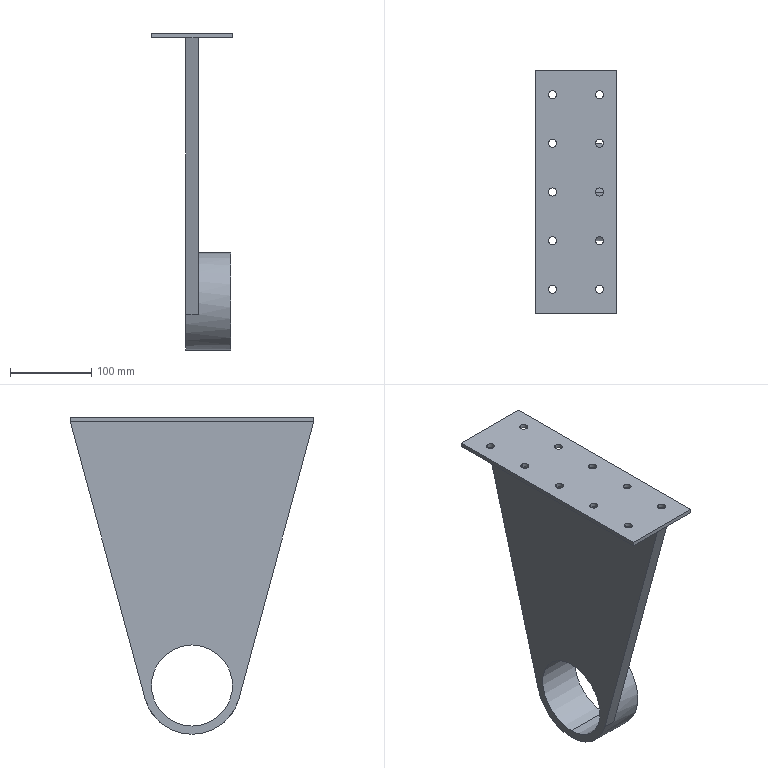Component | SolidWorks | BrushRollerHolder-1 | 1 solid | 36 faces | box 100 x 300 x 390 mm | volume 1352677 mm3 | cylinder 24 | plane 12 | commonest cylinder face diameters 10 x20 100 x2 120 x2
build123d program:
from build123d import *

# Parameters (mm, degrees)
SKETCH1_W                = 300
SKETCH1_H                = 100
BOSS_EXTRUDE1_DEPTH      = 5
BOSS_EXTRUDE2_DEPTH      = 8
BOSS_EXTRUDE2_DEPTH_BACK = 8
SKETCH4_R                = 50
BOSS_EXTRUDE3_START      = 40
SKETCH5_R                = 60
SKETCH5_R_2              = 50
BOSS_EXTRUDE3_DEPTH      = 40
SKETCH6_R                = 5
CUT_EXTRUDE2_DEPTH       = 40
LPATTERN1_COUNT          = 5
LPATTERN1_PITCH          = 60
MIRROR1_COPY_1_SKETCH_R  = 5
MIRROR1_COPY_1_DEPTH     = 40
MIRROR1_COPY_2_SKETCH_R  = 5
MIRROR1_COPY_2_DEPTH     = 40
MIRROR1_COPY_3_SKETCH_R  = 5
MIRROR1_COPY_3_DEPTH     = 40
MIRROR1_COPY_4_SKETCH_R  = 5
MIRROR1_COPY_4_DEPTH     = 40


with BuildPart() as part:
    # Sketch1 → Boss-Extrude1 (new body)
    with BuildSketch(Plane.XY):
        Rectangle(SKETCH1_W, SKETCH1_H)
    extrude(amount=BOSS_EXTRUDE1_DEPTH)

    # Sketch4 → Boss-Extrude2 (add, two sides: drawn at the far end of the back side and taken through both)
    with BuildSketch(Plane(origin=(0, 0, 0), x_dir=(1, 0, 0), z_dir=(0, 1, 0)).offset(-BOSS_EXTRUDE2_DEPTH_BACK)):
        with BuildLine():
            Line((-57.921, 340.656), (-150, 0))
            Line((-150, 0), (150, 0))
            Line((150, 0), (57.921, 340.656))
            ThreePointArc((57.921, 340.656), (0, 385), (-57.921, 340.656))
        make_face()
        with Locations(Location((0, 325, 0), (0, 0, 270))):
            Circle(SKETCH4_R, mode=Mode.SUBTRACT)
    extrude(amount=BOSS_EXTRUDE2_DEPTH + BOSS_EXTRUDE2_DEPTH_BACK)

    # Sketch5 → Boss-Extrude3 (add)
    with BuildSketch(Plane(origin=(0, -8, 0), x_dir=(-1, 0, 0), z_dir=(0, -1, 0)).offset(BOSS_EXTRUDE3_START)):
        with Locations(Location((0, 325, 0), (0, 0, 15.125))):
            Circle(SKETCH5_R)
        with Locations(Location((0, 325, 0), (0, 0, 270))):
            Circle(SKETCH5_R_2, mode=Mode.SUBTRACT)
    extrude(amount=-BOSS_EXTRUDE3_DEPTH)

    # Sketch6 → Cut-Extrude2 (cut)
    with BuildSketch(Plane(origin=(0, 0, 0), x_dir=(-1, 0, 0), z_dir=(0, 0, -1))):
        with Locations((-120, 29)):
            Circle(SKETCH6_R)
    cut_extrude2 = extrude(amount=-CUT_EXTRUDE2_DEPTH, mode=Mode.SUBTRACT)

    # LPattern1: Cut-Extrude2 ×5
    with Locations(*[(-i * LPATTERN1_PITCH, 0, 0) for i in range(1, LPATTERN1_COUNT)]):
        add(cut_extrude2, mode=Mode.SUBTRACT)

    # Mirror1: Cut-Extrude2 across plane
    add(cut_extrude2.mirror(Plane.ZX), mode=Mode.SUBTRACT)

    # Mirror1 copy 1 sketch → Mirror1 copy 1 (cut)
    with BuildSketch(Plane(origin=(-60, 0, 0), x_dir=(-1, 0, 0), z_dir=(0, 0, -1))):
        with Locations((-120, -29)):
            Circle(MIRROR1_COPY_1_SKETCH_R)
    extrude(amount=-MIRROR1_COPY_1_DEPTH, mode=Mode.SUBTRACT)

    # Mirror1 copy 2 sketch → Mirror1 copy 2 (cut)
    with BuildSketch(Plane(origin=(-120, 0, 0), x_dir=(-1, 0, 0), z_dir=(0, 0, -1))):
        with Locations((-120, -29)):
            Circle(MIRROR1_COPY_2_SKETCH_R)
    extrude(amount=-MIRROR1_COPY_2_DEPTH, mode=Mode.SUBTRACT)

    # Mirror1 copy 3 sketch → Mirror1 copy 3 (cut)
    with BuildSketch(Plane(origin=(-180, 0, 0), x_dir=(-1, 0, 0), z_dir=(0, 0, -1))):
        with Locations((-120, -29)):
            Circle(MIRROR1_COPY_3_SKETCH_R)
    extrude(amount=-MIRROR1_COPY_3_DEPTH, mode=Mode.SUBTRACT)

    # Mirror1 copy 4 sketch → Mirror1 copy 4 (cut)
    with BuildSketch(Plane(origin=(-240, 0, 0), x_dir=(-1, 0, 0), z_dir=(0, 0, -1))):
        with Locations((-120, -29)):
            Circle(MIRROR1_COPY_4_SKETCH_R)
    extrude(amount=-MIRROR1_COPY_4_DEPTH, mode=Mode.SUBTRACT)


solid = part.part

# Placed as in the assembly
solid = solid.moved(Location((-316.371, -447.9, 410), (0, 0, 90)))